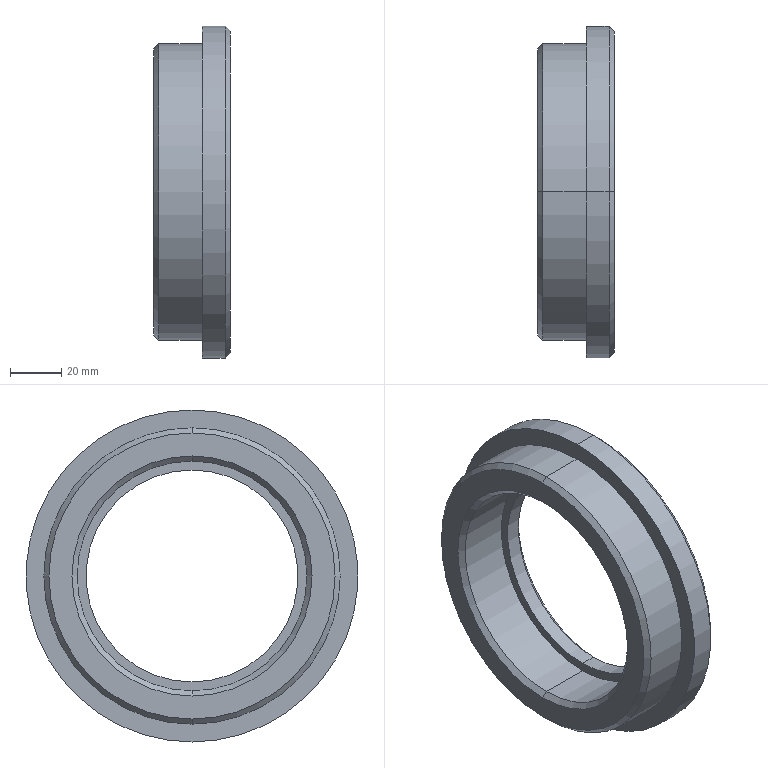Component | SolidWorks | THK-A1004LiftingMotorMountingRoundPlateLeft-1 | 1 solid | 20 faces | box 30 x 130 x 130 mm | volume 160928 mm3 | cone 8 | cylinder 8 | plane 4 | commonest cylinder face diameters 90 x2 116 x2 130 x2 83 x2 | material 45
build123d program:
from build123d import *

# Parameters (mm, degrees)
CHAMFER1_SIZE = 2


with BuildPart() as part:
    # Sketch4 → Revolve1 (revolve)
    with BuildSketch(Plane(origin=(0, 0, 0), x_dir=(1, 0, 0), z_dir=(0, 1, 0)), mode=Mode.PRIVATE) as revolve1_sk:
        Polygon((0, 41.5), (0, 65), (-11, 65), (-11, 58), (-30, 58), (-30, 45), (-8, 45), (-8, 41.5), align=None)
    revolve(revolve1_sk.sketch.rotate(Axis((-49.996, 0, 0), (1, 0, 0)), 180), axis=Axis((-49.996, 0, 0), (1, 0, 0)))

    # Chamfer1
    chamfer1_edges = [part.edges().sort_by_distance(p)[0] for p in [
        (-30, 0, -45),
        (-30, 0, -58),
        (0, 0, -65),
        (0, 0, -41.5),
    ]]
    chamfer(chamfer1_edges, length=CHAMFER1_SIZE)


solid = part.part

# Placed as in the assembly
solid = solid.moved(Location((-105, 383, -155), (0, 0, 0)))
STEP:
#1=CARTESIAN_POINT('',(-5.236,15.079,-7.874));
#2=VERTEX_POINT('',#1);
#3=CARTESIAN_POINT('',(-5.236,15.079,-4.331));
#4=VERTEX_POINT('',#3);
#5=CARTESIAN_POINT('',(-5.236,15.079,-6.102));
#6=DIRECTION('',(-1.,0.,0.));
#7=DIRECTION('',(0.,0.,-1.));
#8=AXIS2_PLACEMENT_3D('',#5,#6,#7);
#9=CIRCLE('',#8,1.772);
#10=EDGE_CURVE('',#2,#4,#9,.T.);
#11=ORIENTED_EDGE('',*,*,#10,.F.);
#12=CARTESIAN_POINT('',(-5.315,15.079,-7.953));
#13=VERTEX_POINT('',#12);
#14=CARTESIAN_POINT('',(-5.236,15.079,-7.874));
#15=DIRECTION('',(-0.7071,0.,-0.7071));
#16=VECTOR('',#15,39.37);
#17=LINE('',#14,#16);
#18=EDGE_CURVE('',#2,#13,#17,.T.);
#19=ORIENTED_EDGE('',*,*,#18,.T.);
#20=CARTESIAN_POINT('',(-5.315,15.079,-4.252));
#21=VERTEX_POINT('',#20);
#22=CARTESIAN_POINT('',(-5.315,15.079,-6.102));
#23=DIRECTION('',(1.,0.,0.));
#24=DIRECTION('',(0.,0.,-1.));
#25=AXIS2_PLACEMENT_3D('',#22,#23,#24);
#26=CIRCLE('',#25,1.85);
#27=EDGE_CURVE('',#21,#13,#26,.T.);
#28=ORIENTED_EDGE('',*,*,#27,.F.);
#29=CARTESIAN_POINT('',(-5.236,15.079,-4.331));
#30=DIRECTION('',(-0.7071,0.,0.7071));
#31=VECTOR('',#30,39.37);
#32=LINE('',#29,#31);
#33=EDGE_CURVE('',#4,#21,#32,.T.);
#34=ORIENTED_EDGE('',*,*,#33,.F.);
#35=EDGE_LOOP('',(#11,#19,#28,#34));
#36=FACE_OUTER_BOUND('',#35,.T.);
#37=CARTESIAN_POINT('',(-5.236,15.079,-6.102));
#38=DIRECTION('',(-1.,0.,0.));
#39=DIRECTION('',(0.,0.,1.));
#40=AXIS2_PLACEMENT_3D('',#37,#38,#39);
#41=CONICAL_SURFACE('',#40,1.772,0.7854);
#42=ADVANCED_FACE('',(#36),#41,.F.);
#43=CARTESIAN_POINT('',(-5.315,15.079,-3.898));
#44=VERTEX_POINT('',#43);
#45=CARTESIAN_POINT('',(-5.315,15.079,-8.307));
#46=VERTEX_POINT('',#45);
#47=CARTESIAN_POINT('',(-5.315,15.079,-6.102));
#48=DIRECTION('',(-1.,0.,0.));
#49=DIRECTION('',(0.,0.,-1.));
#50=AXIS2_PLACEMENT_3D('',#47,#48,#49);
#51=CIRCLE('',#50,2.205);
#52=EDGE_CURVE('',#44,#46,#51,.T.);
#53=ORIENTED_EDGE('',*,*,#52,.F.);
#54=CARTESIAN_POINT('',(-5.236,15.079,-3.819));
#55=VERTEX_POINT('',#54);
#56=CARTESIAN_POINT('',(-5.315,15.079,-3.898));
#57=DIRECTION('',(0.7071,0.,0.7071));
#58=VECTOR('',#57,39.37);
#59=LINE('',#56,#58);
#60=EDGE_CURVE('',#44,#55,#59,.T.);
#61=ORIENTED_EDGE('',*,*,#60,.T.);
#62=CARTESIAN_POINT('',(-5.236,15.079,-8.386));
#63=VERTEX_POINT('',#62);
#64=CARTESIAN_POINT('',(-5.236,15.079,-6.102));
#65=DIRECTION('',(1.,0.,0.));
#66=DIRECTION('',(0.,0.,-1.));
#67=AXIS2_PLACEMENT_3D('',#64,#65,#66);
#68=CIRCLE('',#67,2.283);
#69=EDGE_CURVE('',#63,#55,#68,.T.);
#70=ORIENTED_EDGE('',*,*,#69,.F.);
#71=CARTESIAN_POINT('',(-5.315,15.079,-8.307));
#72=DIRECTION('',(0.7071,0.,-0.7071));
#73=VECTOR('',#72,39.37);
#74=LINE('',#71,#73);
#75=EDGE_CURVE('',#46,#63,#74,.T.);
#76=ORIENTED_EDGE('',*,*,#75,.F.);
#77=EDGE_LOOP('',(#53,#61,#70,#76));
#78=FACE_OUTER_BOUND('',#77,.T.);
#79=CARTESIAN_POINT('',(-5.315,15.079,-6.102));
#80=DIRECTION('',(1.,0.,0.));
#81=DIRECTION('',(0.,0.,-1.));
#82=AXIS2_PLACEMENT_3D('',#79,#80,#81);
#83=CONICAL_SURFACE('',#82,2.205,0.7854);
#84=ADVANCED_FACE('',(#78),#83,.T.);
#85=CARTESIAN_POINT('',(-4.213,15.079,-4.469));
#86=VERTEX_POINT('',#85);
#87=CARTESIAN_POINT('',(-4.213,15.079,-7.736));
#88=VERTEX_POINT('',#87);
#89=CARTESIAN_POINT('',(-4.213,15.079,-6.102));
#90=DIRECTION('',(1.,0.,0.));
#91=DIRECTION('',(0.,0.,1.));
#92=AXIS2_PLACEMENT_3D('',#89,#90,#91);
#93=CIRCLE('',#92,1.634);
#94=EDGE_CURVE('',#86,#88,#93,.T.);
#95=ORIENTED_EDGE('',*,*,#94,.F.);
#96=CARTESIAN_POINT('',(-4.134,15.079,-4.39));
#97=VERTEX_POINT('',#96);
#98=CARTESIAN_POINT('',(-4.134,15.079,-4.39));
#99=DIRECTION('',(0.7071,0.,0.7071));
#100=VECTOR('',#99,39.37);
#101=LINE('',#98,#100);
#102=EDGE_CURVE('',#86,#97,#101,.T.);
#103=ORIENTED_EDGE('',*,*,#102,.T.);
#104=CARTESIAN_POINT('',(-4.134,15.079,-7.815));
#105=VERTEX_POINT('',#104);
#106=CARTESIAN_POINT('',(-4.134,15.079,-6.102));
#107=DIRECTION('',(-1.,0.,0.));
#108=DIRECTION('',(0.,0.,1.));
#109=AXIS2_PLACEMENT_3D('',#106,#107,#108);
#110=CIRCLE('',#109,1.713);
#111=EDGE_CURVE('',#105,#97,#110,.T.);
#112=ORIENTED_EDGE('',*,*,#111,.F.);
#113=CARTESIAN_POINT('',(-4.134,15.079,-7.815));
#114=DIRECTION('',(0.7071,0.,-0.7071));
#115=VECTOR('',#114,39.37);
#116=LINE('',#113,#115);
#117=EDGE_CURVE('',#88,#105,#116,.T.);
#118=ORIENTED_EDGE('',*,*,#117,.F.);
#119=EDGE_LOOP('',(#95,#103,#112,#118));
#120=FACE_OUTER_BOUND('',#119,.T.);
#121=CARTESIAN_POINT('',(-4.134,15.079,-6.102));
#122=DIRECTION('',(1.,0.,0.));
#123=DIRECTION('',(0.,0.,-1.));
#124=AXIS2_PLACEMENT_3D('',#121,#122,#123);
#125=CONICAL_SURFACE('',#124,1.713,0.7854);
#126=ADVANCED_FACE('',(#120),#125,.F.);
#127=CARTESIAN_POINT('',(-4.134,15.079,-8.583));
#128=VERTEX_POINT('',#127);
#129=CARTESIAN_POINT('',(-4.134,15.079,-3.622));
#130=VERTEX_POINT('',#129);
#131=CARTESIAN_POINT('',(-4.134,15.079,-6.102));
#132=DIRECTION('',(1.,0.,0.));
#133=DIRECTION('',(0.,0.,1.));
#134=AXIS2_PLACEMENT_3D('',#131,#132,#133);
#135=CIRCLE('',#134,2.48);
#136=EDGE_CURVE('',#128,#130,#135,.T.);
#137=ORIENTED_EDGE('',*,*,#136,.F.);
#138=CARTESIAN_POINT('',(-4.213,15.079,-8.661));
#139=VERTEX_POINT('',#138);
#140=CARTESIAN_POINT('',(-4.213,15.079,-8.661));
#141=DIRECTION('',(-0.7071,0.,-0.7071));
#142=VECTOR('',#141,39.37);
#143=LINE('',#140,#142);
#144=EDGE_CURVE('',#128,#139,#143,.T.);
#145=ORIENTED_EDGE('',*,*,#144,.T.);
#146=CARTESIAN_POINT('',(-4.213,15.079,-3.543));
#147=VERTEX_POINT('',#146);
#148=CARTESIAN_POINT('',(-4.213,15.079,-6.102));
#149=DIRECTION('',(-1.,0.,0.));
#150=DIRECTION('',(0.,0.,1.));
#151=AXIS2_PLACEMENT_3D('',#148,#149,#150);
#152=CIRCLE('',#151,2.559);
#153=EDGE_CURVE('',#147,#139,#152,.T.);
#154=ORIENTED_EDGE('',*,*,#153,.F.);
#155=CARTESIAN_POINT('',(-4.213,15.079,-3.543));
#156=DIRECTION('',(-0.7071,0.,0.7071));
#157=VECTOR('',#156,39.37);
#158=LINE('',#155,#157);
#159=EDGE_CURVE('',#130,#147,#158,.T.);
#160=ORIENTED_EDGE('',*,*,#159,.F.);
#161=EDGE_LOOP('',(#137,#145,#154,#160));
#162=FACE_OUTER_BOUND('',#161,.T.);
#163=CARTESIAN_POINT('',(-4.213,15.079,-6.102));
#164=DIRECTION('',(-1.,0.,0.));
#165=DIRECTION('',(0.,0.,1.));
#166=AXIS2_PLACEMENT_3D('',#163,#164,#165);
#167=CONICAL_SURFACE('',#166,2.559,0.7854);
#168=ADVANCED_FACE('',(#162),#167,.T.);
#169=CARTESIAN_POINT('',(-4.449,15.079,-7.874));
#170=VERTEX_POINT('',#169);
#171=CARTESIAN_POINT('',(-4.449,15.079,-4.331));
#172=VERTEX_POINT('',#171);
#173=CARTESIAN_POINT('',(-4.449,15.079,-6.102));
#174=DIRECTION('',(-1.,0.,0.));
#175=DIRECTION('',(0.,0.,1.));
#176=AXIS2_PLACEMENT_3D('',#173,#174,#175);
#177=CIRCLE('',#176,1.772);
#178=EDGE_CURVE('',#170,#172,#177,.T.);
#179=ORIENTED_EDGE('',*,*,#178,.F.);
#180=CARTESIAN_POINT('',(-6.102,15.079,-7.874));
#181=DIRECTION('',(-1.,0.,0.));
#182=VECTOR('',#181,39.37);
#183=LINE('',#180,#182);
#184=EDGE_CURVE('',#170,#2,#183,.T.);
#185=ORIENTED_EDGE('',*,*,#184,.T.);
#186=ORIENTED_EDGE('',*,*,#10,.T.);
#187=CARTESIAN_POINT('',(-6.102,15.079,-4.331));
#188=DIRECTION('',(-1.,0.,0.));
#189=VECTOR('',#188,39.37);
#190=LINE('',#187,#189);
#191=EDGE_CURVE('',#172,#4,#190,.T.);
#192=ORIENTED_EDGE('',*,*,#191,.F.);
#193=EDGE_LOOP('',(#179,#185,#186,#192));
#194=FACE_OUTER_BOUND('',#193,.T.);
#195=CARTESIAN_POINT('',(-6.102,15.079,-6.102));
#196=DIRECTION('',(-1.,0.,0.));
#197=DIRECTION('',(0.,0.,1.));
#198=AXIS2_PLACEMENT_3D('',#195,#196,#197);
#199=CYLINDRICAL_SURFACE('',#198,1.772);
#200=ADVANCED_FACE('',(#194),#199,.F.);
#201=CARTESIAN_POINT('',(-4.567,15.079,-3.819));
#202=VERTEX_POINT('',#201);
#203=CARTESIAN_POINT('',(-4.567,15.079,-8.386));
#204=VERTEX_POINT('',#203);
#205=CARTESIAN_POINT('',(-4.567,15.079,-6.102));
#206=DIRECTION('',(-1.,0.,0.));
#207=DIRECTION('',(0.,0.,1.));
#208=AXIS2_PLACEMENT_3D('',#205,#206,#207);
#209=CIRCLE('',#208,2.283);
#210=EDGE_CURVE('',#202,#204,#209,.T.);
#211=ORIENTED_EDGE('',*,*,#210,.T.);
#212=CARTESIAN_POINT('',(-6.102,15.079,-8.386));
#213=DIRECTION('',(-1.,0.,0.));
#214=VECTOR('',#213,39.37);
#215=LINE('',#212,#214);
#216=EDGE_CURVE('',#204,#63,#215,.T.);
#217=ORIENTED_EDGE('',*,*,#216,.T.);
#218=ORIENTED_EDGE('',*,*,#69,.T.);
#219=CARTESIAN_POINT('',(-6.102,15.079,-3.819));
#220=DIRECTION('',(-1.,0.,0.));
#221=VECTOR('',#220,39.37);
#222=LINE('',#219,#221);
#223=EDGE_CURVE('',#202,#55,#222,.T.);
#224=ORIENTED_EDGE('',*,*,#223,.F.);
#225=EDGE_LOOP('',(#211,#217,#218,#224));
#226=FACE_OUTER_BOUND('',#225,.T.);
#227=CARTESIAN_POINT('',(-6.102,15.079,-6.102));
#228=DIRECTION('',(-1.,0.,0.));
#229=DIRECTION('',(0.,0.,1.));
#230=AXIS2_PLACEMENT_3D('',#227,#228,#229);
#231=CYLINDRICAL_SURFACE('',#230,2.283);
#232=ADVANCED_FACE('',(#226),#231,.T.);
#233=ORIENTED_EDGE('',*,*,#153,.T.);
#234=CARTESIAN_POINT('',(-4.567,15.079,-8.661));
#235=VERTEX_POINT('',#234);
#236=CARTESIAN_POINT('',(-6.102,15.079,-8.661));
#237=DIRECTION('',(-1.,0.,0.));
#238=VECTOR('',#237,39.37);
#239=LINE('',#236,#238);
#240=EDGE_CURVE('',#139,#235,#239,.T.);
#241=ORIENTED_EDGE('',*,*,#240,.T.);
#242=CARTESIAN_POINT('',(-4.567,15.079,-3.543));
#243=VERTEX_POINT('',#242);
#244=CARTESIAN_POINT('',(-4.567,15.079,-6.102));
#245=DIRECTION('',(-1.,0.,0.));
#246=DIRECTION('',(0.,0.,1.));
#247=AXIS2_PLACEMENT_3D('',#244,#245,#246);
#248=CIRCLE('',#247,2.559);
#249=EDGE_CURVE('',#243,#235,#248,.T.);
#250=ORIENTED_EDGE('',*,*,#249,.F.);
#251=CARTESIAN_POINT('',(-6.102,15.079,-3.543));
#252=DIRECTION('',(-1.,0.,0.));
#253=VECTOR('',#252,39.37);
#254=LINE('',#251,#253);
#255=EDGE_CURVE('',#147,#243,#254,.T.);
#256=ORIENTED_EDGE('',*,*,#255,.F.);
#257=EDGE_LOOP('',(#233,#241,#250,#256));
#258=FACE_OUTER_BOUND('',#257,.T.);
#259=CARTESIAN_POINT('',(-6.102,15.079,-6.102));
#260=DIRECTION('',(-1.,0.,0.));
#261=DIRECTION('',(0.,0.,1.));
#262=AXIS2_PLACEMENT_3D('',#259,#260,#261);
#263=CYLINDRICAL_SURFACE('',#262,2.559);
#264=ADVANCED_FACE('',(#258),#263,.T.);
#265=ORIENTED_EDGE('',*,*,#94,.T.);
#266=CARTESIAN_POINT('',(-4.449,15.079,-7.736));
#267=VERTEX_POINT('',#266);
#268=CARTESIAN_POINT('',(-6.102,15.079,-7.736));
#269=DIRECTION('',(-1.,0.,0.));
#270=VECTOR('',#269,39.37);
#271=LINE('',#268,#270);
#272=EDGE_CURVE('',#88,#267,#271,.T.);
#273=ORIENTED_EDGE('',*,*,#272,.T.);
#274=CARTESIAN_POINT('',(-4.449,15.079,-4.469));
#275=VERTEX_POINT('',#274);
#276=CARTESIAN_POINT('',(-4.449,15.079,-6.102));
#277=DIRECTION('',(-1.,0.,0.));
#278=DIRECTION('',(0.,0.,1.));
#279=AXIS2_PLACEMENT_3D('',#276,#277,#278);
#280=CIRCLE('',#279,1.634);
#281=EDGE_CURVE('',#267,#275,#280,.T.);
#282=ORIENTED_EDGE('',*,*,#281,.T.);
#283=CARTESIAN_POINT('',(-6.102,15.079,-4.469));
#284=DIRECTION('',(-1.,0.,0.));
#285=VECTOR('',#284,39.37);
#286=LINE('',#283,#285);
#287=EDGE_CURVE('',#86,#275,#286,.T.);
#288=ORIENTED_EDGE('',*,*,#287,.F.);
#289=EDGE_LOOP('',(#265,#273,#282,#288));
#290=FACE_OUTER_BOUND('',#289,.T.);
#291=CARTESIAN_POINT('',(-6.102,15.079,-6.102));
#292=DIRECTION('',(-1.,0.,0.));
#293=DIRECTION('',(0.,0.,1.));
#294=AXIS2_PLACEMENT_3D('',#291,#292,#293);
#295=CYLINDRICAL_SURFACE('',#294,1.634);
#296=ADVANCED_FACE('',(#290),#295,.F.);
#297=ORIENTED_EDGE('',*,*,#272,.F.);
#298=CARTESIAN_POINT('',(-4.213,15.079,-6.102));
#299=DIRECTION('',(1.,0.,0.));
#300=DIRECTION('',(0.,0.,1.));
#301=AXIS2_PLACEMENT_3D('',#298,#299,#300);
#302=CIRCLE('',#301,1.634);
#303=EDGE_CURVE('',#88,#86,#302,.T.);
#304=ORIENTED_EDGE('',*,*,#303,.T.);
#305=ORIENTED_EDGE('',*,*,#287,.T.);
#306=CARTESIAN_POINT('',(-4.449,15.079,-6.102));
#307=DIRECTION('',(-1.,0.,0.));
#308=DIRECTION('',(0.,0.,1.));
#309=AXIS2_PLACEMENT_3D('',#306,#307,#308);
#310=CIRCLE('',#309,1.634);
#311=EDGE_CURVE('',#275,#267,#310,.T.);
#312=ORIENTED_EDGE('',*,*,#311,.T.);
#313=EDGE_LOOP('',(#297,#304,#305,#312));
#314=FACE_OUTER_BOUND('',#313,.T.);
#315=CARTESIAN_POINT('',(-6.102,15.079,-6.102));
#316=DIRECTION('',(-1.,0.,0.));
#317=DIRECTION('',(0.,0.,1.));
#318=AXIS2_PLACEMENT_3D('',#315,#316,#317);
#319=CYLINDRICAL_SURFACE('',#318,1.634);
#320=ADVANCED_FACE('',(#314),#319,.F.);
#321=CARTESIAN_POINT('',(-4.134,15.079,-6.102));
#322=DIRECTION('',(1.,0.,0.));
#323=DIRECTION('',(0.,0.,1.));
#324=AXIS2_PLACEMENT_3D('',#321,#322,#323);
#325=CIRCLE('',#324,2.48);
#326=EDGE_CURVE('',#130,#128,#325,.T.);
#327=ORIENTED_EDGE('',*,*,#326,.T.);
#328=ORIENTED_EDGE('',*,*,#136,.T.);
#329=EDGE_LOOP('',(#327,#328));
#330=FACE_OUTER_BOUND('',#329,.T.);
#331=ORIENTED_EDGE('',*,*,#111,.T.);
#332=CARTESIAN_POINT('',(-4.134,15.079,-6.102));
#333=DIRECTION('',(-1.,0.,0.));
#334=DIRECTION('',(0.,0.,1.));
#335=AXIS2_PLACEMENT_3D('',#332,#333,#334);
#336=CIRCLE('',#335,1.713);
#337=EDGE_CURVE('',#97,#105,#336,.T.);
#338=ORIENTED_EDGE('',*,*,#337,.T.);
#339=EDGE_LOOP('',(#331,#338));
#340=FACE_BOUND('',#339,.T.);
#341=CARTESIAN_POINT('',(-4.134,15.079,-7.736));
#342=DIRECTION('',(-1.,0.,0.));
#343=DIRECTION('',(0.,0.,1.));
#344=AXIS2_PLACEMENT_3D('',#341,#342,#343);
#345=PLANE('',#344);
#346=ADVANCED_FACE('',(#330,#340),#345,.F.);
#347=ORIENTED_EDGE('',*,*,#240,.F.);
#348=CARTESIAN_POINT('',(-4.213,15.079,-6.102));
#349=DIRECTION('',(-1.,0.,0.));
#350=DIRECTION('',(0.,0.,1.));
#351=AXIS2_PLACEMENT_3D('',#348,#349,#350);
#352=CIRCLE('',#351,2.559);
#353=EDGE_CURVE('',#139,#147,#352,.T.);
#354=ORIENTED_EDGE('',*,*,#353,.T.);
#355=ORIENTED_EDGE('',*,*,#255,.T.);
#356=CARTESIAN_POINT('',(-4.567,15.079,-6.102));
#357=DIRECTION('',(-1.,0.,0.));
#358=DIRECTION('',(0.,0.,1.));
#359=AXIS2_PLACEMENT_3D('',#356,#357,#358);
#360=CIRCLE('',#359,2.559);
#361=EDGE_CURVE('',#235,#243,#360,.T.);
#362=ORIENTED_EDGE('',*,*,#361,.F.);
#363=EDGE_LOOP('',(#347,#354,#355,#362));
#364=FACE_OUTER_BOUND('',#363,.T.);
#365=CARTESIAN_POINT('',(-6.102,15.079,-6.102));
#366=DIRECTION('',(-1.,0.,0.));
#367=DIRECTION('',(0.,0.,1.));
#368=AXIS2_PLACEMENT_3D('',#365,#366,#367);
#369=CYLINDRICAL_SURFACE('',#368,2.559);
#370=ADVANCED_FACE('',(#364),#369,.T.);
#371=ORIENTED_EDGE('',*,*,#210,.F.);
#372=CARTESIAN_POINT('',(-4.567,15.079,-6.102));
#373=DIRECTION('',(-1.,0.,0.));
#374=DIRECTION('',(0.,0.,1.));
#375=AXIS2_PLACEMENT_3D('',#372,#373,#374);
#376=CIRCLE('',#375,2.283);
#377=EDGE_CURVE('',#204,#202,#376,.T.);
#378=ORIENTED_EDGE('',*,*,#377,.F.);
#379=EDGE_LOOP('',(#371,#378));
#380=FACE_BOUND('',#379,.T.);
#381=ORIENTED_EDGE('',*,*,#249,.T.);
#382=ORIENTED_EDGE('',*,*,#361,.T.);
#383=EDGE_LOOP('',(#381,#382));
#384=FACE_OUTER_BOUND('',#383,.T.);
#385=CARTESIAN_POINT('',(-4.567,15.079,-8.661));
#386=DIRECTION('',(1.,0.,0.));
#387=DIRECTION('',(0.,0.,-1.));
#388=AXIS2_PLACEMENT_3D('',#385,#386,#387);
#389=PLANE('',#388);
#390=ADVANCED_FACE('',(#380,#384),#389,.F.);
#391=ORIENTED_EDGE('',*,*,#216,.F.);
#392=ORIENTED_EDGE('',*,*,#377,.T.);
#393=ORIENTED_EDGE('',*,*,#223,.T.);
#394=CARTESIAN_POINT('',(-5.236,15.079,-6.102));
#395=DIRECTION('',(1.,0.,0.));
#396=DIRECTION('',(0.,0.,-1.));
#397=AXIS2_PLACEMENT_3D('',#394,#395,#396);
#398=CIRCLE('',#397,2.283);
#399=EDGE_CURVE('',#55,#63,#398,.T.);
#400=ORIENTED_EDGE('',*,*,#399,.T.);
#401=EDGE_LOOP('',(#391,#392,#393,#400));
#402=FACE_OUTER_BOUND('',#401,.T.);
#403=CARTESIAN_POINT('',(-6.102,15.079,-6.102));
#404=DIRECTION('',(-1.,0.,0.));
#405=DIRECTION('',(0.,0.,1.));
#406=AXIS2_PLACEMENT_3D('',#403,#404,#405);
#407=CYLINDRICAL_SURFACE('',#406,2.283);
#408=ADVANCED_FACE('',(#402),#407,.T.);
#409=CARTESIAN_POINT('',(-5.315,15.079,-6.102));
#410=DIRECTION('',(-1.,0.,0.));
#411=DIRECTION('',(0.,0.,-1.));
#412=AXIS2_PLACEMENT_3D('',#409,#410,#411);
#413=CIRCLE('',#412,2.205);
#414=EDGE_CURVE('',#46,#44,#413,.T.);
#415=ORIENTED_EDGE('',*,*,#414,.T.);
#416=ORIENTED_EDGE('',*,*,#52,.T.);
#417=EDGE_LOOP('',(#415,#416));
#418=FACE_OUTER_BOUND('',#417,.T.);
#419=ORIENTED_EDGE('',*,*,#27,.T.);
#420=CARTESIAN_POINT('',(-5.315,15.079,-6.102));
#421=DIRECTION('',(1.,0.,0.));
#422=DIRECTION('',(0.,0.,-1.));
#423=AXIS2_PLACEMENT_3D('',#420,#421,#422);
#424=CIRCLE('',#423,1.85);
#425=EDGE_CURVE('',#13,#21,#424,.T.);
#426=ORIENTED_EDGE('',*,*,#425,.T.);
#427=EDGE_LOOP('',(#419,#426));
#428=FACE_BOUND('',#427,.T.);
#429=CARTESIAN_POINT('',(-5.315,15.079,-8.386));
#430=DIRECTION('',(1.,0.,0.));
#431=DIRECTION('',(0.,0.,-1.));
#432=AXIS2_PLACEMENT_3D('',#429,#430,#431);
#433=PLANE('',#432);
#434=ADVANCED_FACE('',(#418,#428),#433,.F.);
#435=ORIENTED_EDGE('',*,*,#184,.F.);
#436=CARTESIAN_POINT('',(-4.449,15.079,-6.102));
#437=DIRECTION('',(-1.,0.,0.));
#438=DIRECTION('',(0.,0.,1.));
#439=AXIS2_PLACEMENT_3D('',#436,#437,#438);
#440=CIRCLE('',#439,1.772);
#441=EDGE_CURVE('',#172,#170,#440,.T.);
#442=ORIENTED_EDGE('',*,*,#441,.F.);
#443=ORIENTED_EDGE('',*,*,#191,.T.);
#444=CARTESIAN_POINT('',(-5.236,15.079,-6.102));
#445=DIRECTION('',(-1.,0.,0.));
#446=DIRECTION('',(0.,0.,-1.));
#447=AXIS2_PLACEMENT_3D('',#444,#445,#446);
#448=CIRCLE('',#447,1.772);
#449=EDGE_CURVE('',#4,#2,#448,.T.);
#450=ORIENTED_EDGE('',*,*,#449,.T.);
#451=EDGE_LOOP('',(#435,#442,#443,#450));
#452=FACE_OUTER_BOUND('',#451,.T.);
#453=CARTESIAN_POINT('',(-6.102,15.079,-6.102));
#454=DIRECTION('',(-1.,0.,0.));
#455=DIRECTION('',(0.,0.,1.));
#456=AXIS2_PLACEMENT_3D('',#453,#454,#455);
#457=CYLINDRICAL_SURFACE('',#456,1.772);
#458=ADVANCED_FACE('',(#452),#457,.F.);
#459=ORIENTED_EDGE('',*,*,#311,.F.);
#460=ORIENTED_EDGE('',*,*,#281,.F.);
#461=EDGE_LOOP('',(#459,#460));
#462=FACE_BOUND('',#461,.T.);
#463=ORIENTED_EDGE('',*,*,#441,.T.);
#464=ORIENTED_EDGE('',*,*,#178,.T.);
#465=EDGE_LOOP('',(#463,#464));
#466=FACE_OUTER_BOUND('',#465,.T.);
#467=CARTESIAN_POINT('',(-4.449,15.079,-7.874));
#468=DIRECTION('',(1.,0.,0.));
#469=DIRECTION('',(0.,0.,-1.));
#470=AXIS2_PLACEMENT_3D('',#467,#468,#469);
#471=PLANE('',#470);
#472=ADVANCED_FACE('',(#462,#466),#471,.F.);
#473=ORIENTED_EDGE('',*,*,#144,.F.);
#474=ORIENTED_EDGE('',*,*,#326,.F.);
#475=ORIENTED_EDGE('',*,*,#159,.T.);
#476=ORIENTED_EDGE('',*,*,#353,.F.);
#477=EDGE_LOOP('',(#473,#474,#475,#476));
#478=FACE_OUTER_BOUND('',#477,.T.);
#479=CARTESIAN_POINT('',(-4.213,15.079,-6.102));
#480=DIRECTION('',(-1.,0.,0.));
#481=DIRECTION('',(0.,0.,1.));
#482=AXIS2_PLACEMENT_3D('',#479,#480,#481);
#483=CONICAL_SURFACE('',#482,2.559,0.7854);
#484=ADVANCED_FACE('',(#478),#483,.T.);
#485=ORIENTED_EDGE('',*,*,#102,.F.);
#486=ORIENTED_EDGE('',*,*,#303,.F.);
#487=ORIENTED_EDGE('',*,*,#117,.T.);
#488=ORIENTED_EDGE('',*,*,#337,.F.);
#489=EDGE_LOOP('',(#485,#486,#487,#488));
#490=FACE_OUTER_BOUND('',#489,.T.);
#491=CARTESIAN_POINT('',(-4.134,15.079,-6.102));
#492=DIRECTION('',(1.,0.,0.));
#493=DIRECTION('',(0.,0.,-1.));
#494=AXIS2_PLACEMENT_3D('',#491,#492,#493);
#495=CONICAL_SURFACE('',#494,1.713,0.7854);
#496=ADVANCED_FACE('',(#490),#495,.F.);
#497=ORIENTED_EDGE('',*,*,#60,.F.);
#498=ORIENTED_EDGE('',*,*,#414,.F.);
#499=ORIENTED_EDGE('',*,*,#75,.T.);
#500=ORIENTED_EDGE('',*,*,#399,.F.);
#501=EDGE_LOOP('',(#497,#498,#499,#500));
#502=FACE_OUTER_BOUND('',#501,.T.);
#503=CARTESIAN_POINT('',(-5.315,15.079,-6.102));
#504=DIRECTION('',(1.,0.,0.));
#505=DIRECTION('',(0.,0.,-1.));
#506=AXIS2_PLACEMENT_3D('',#503,#504,#505);
#507=CONICAL_SURFACE('',#506,2.205,0.7854);
#508=ADVANCED_FACE('',(#502),#507,.T.);
#509=ORIENTED_EDGE('',*,*,#18,.F.);
#510=ORIENTED_EDGE('',*,*,#449,.F.);
#511=ORIENTED_EDGE('',*,*,#33,.T.);
#512=ORIENTED_EDGE('',*,*,#425,.F.);
#513=EDGE_LOOP('',(#509,#510,#511,#512));
#514=FACE_OUTER_BOUND('',#513,.T.);
#515=CARTESIAN_POINT('',(-5.236,15.079,-6.102));
#516=DIRECTION('',(-1.,0.,0.));
#517=DIRECTION('',(0.,0.,1.));
#518=AXIS2_PLACEMENT_3D('',#515,#516,#517);
#519=CONICAL_SURFACE('',#518,1.772,0.7854);
#520=ADVANCED_FACE('',(#514),#519,.F.);
#521=CLOSED_SHELL('',(#42,#84,#126,#168,#200,#232,#264,#296,#320,#346,#370,#390,#408,#434,#458,#472,#484,#496,#508,#520));
#522=MANIFOLD_SOLID_BREP('',#521);
#523=CARTESIAN_POINT('',(0.,0.,0.));
#524=DIRECTION('',(0.,0.,1.));
#525=DIRECTION('',(1.,0.,0.));
#526=AXIS2_PLACEMENT_3D('',#523,#524,#525);
#527=(LENGTH_UNIT()NAMED_UNIT(*)SI_UNIT($,.METRE.));
#528=LENGTH_MEASURE_WITH_UNIT(LENGTH_MEASURE(0.0254),#527);
#529=DIMENSIONAL_EXPONENTS(1.,0.,0.,0.,0.,0.,0.);
#530=(CONVERSION_BASED_UNIT('',#528)LENGTH_UNIT()NAMED_UNIT(#529));
#531=UNCERTAINTY_MEASURE_WITH_UNIT(LENGTH_MEASURE(0.00001),#530,'','');
#532=(NAMED_UNIT(*)PLANE_ANGLE_UNIT()SI_UNIT($,.RADIAN.));
#533=(NAMED_UNIT(*)SI_UNIT($,.STERADIAN.)SOLID_ANGLE_UNIT());
#534=(GEOMETRIC_REPRESENTATION_CONTEXT(3)GLOBAL_UNCERTAINTY_ASSIGNED_CONTEXT((#531))GLOBAL_UNIT_ASSIGNED_CONTEXT((#530,#532,#533))REPRESENTATION_CONTEXT('',''));
#535=ADVANCED_BREP_SHAPE_REPRESENTATION('',(#522,#526),#534);
#536=COLOUR_RGB('',0.7922,0.8196,0.9333);
#537=FILL_AREA_STYLE_COLOUR('',#536);
#538=FILL_AREA_STYLE('',(#537));
#539=SURFACE_STYLE_FILL_AREA(#538);
#540=SURFACE_SIDE_STYLE('',(#539));
#541=SURFACE_STYLE_USAGE(.BOTH.,#540);
#542=PRESENTATION_STYLE_ASSIGNMENT((#541));
#543=STYLED_ITEM('',(#542),#522);
#544=PRESENTATION_LAYER_ASSIGNMENT('','',(#543));
#545=(LENGTH_UNIT()NAMED_UNIT(*)SI_UNIT($,.METRE.));
#546=LENGTH_MEASURE_WITH_UNIT(LENGTH_MEASURE(0.0254),#545);
#547=DIMENSIONAL_EXPONENTS(1.,0.,0.,0.,0.,0.,0.);
#548=(CONVERSION_BASED_UNIT('',#546)LENGTH_UNIT()NAMED_UNIT(#547));
#549=UNCERTAINTY_MEASURE_WITH_UNIT(LENGTH_MEASURE(0.00001),#548,'','');
#550=(NAMED_UNIT(*)PLANE_ANGLE_UNIT()SI_UNIT($,.RADIAN.));
#551=(NAMED_UNIT(*)SI_UNIT($,.STERADIAN.)SOLID_ANGLE_UNIT());
#552=(GEOMETRIC_REPRESENTATION_CONTEXT(3)GLOBAL_UNCERTAINTY_ASSIGNED_CONTEXT((#549))GLOBAL_UNIT_ASSIGNED_CONTEXT((#548,#550,#551))REPRESENTATION_CONTEXT('',''));
#553=MECHANICAL_DESIGN_GEOMETRIC_PRESENTATION_REPRESENTATION('',(#543),#552);